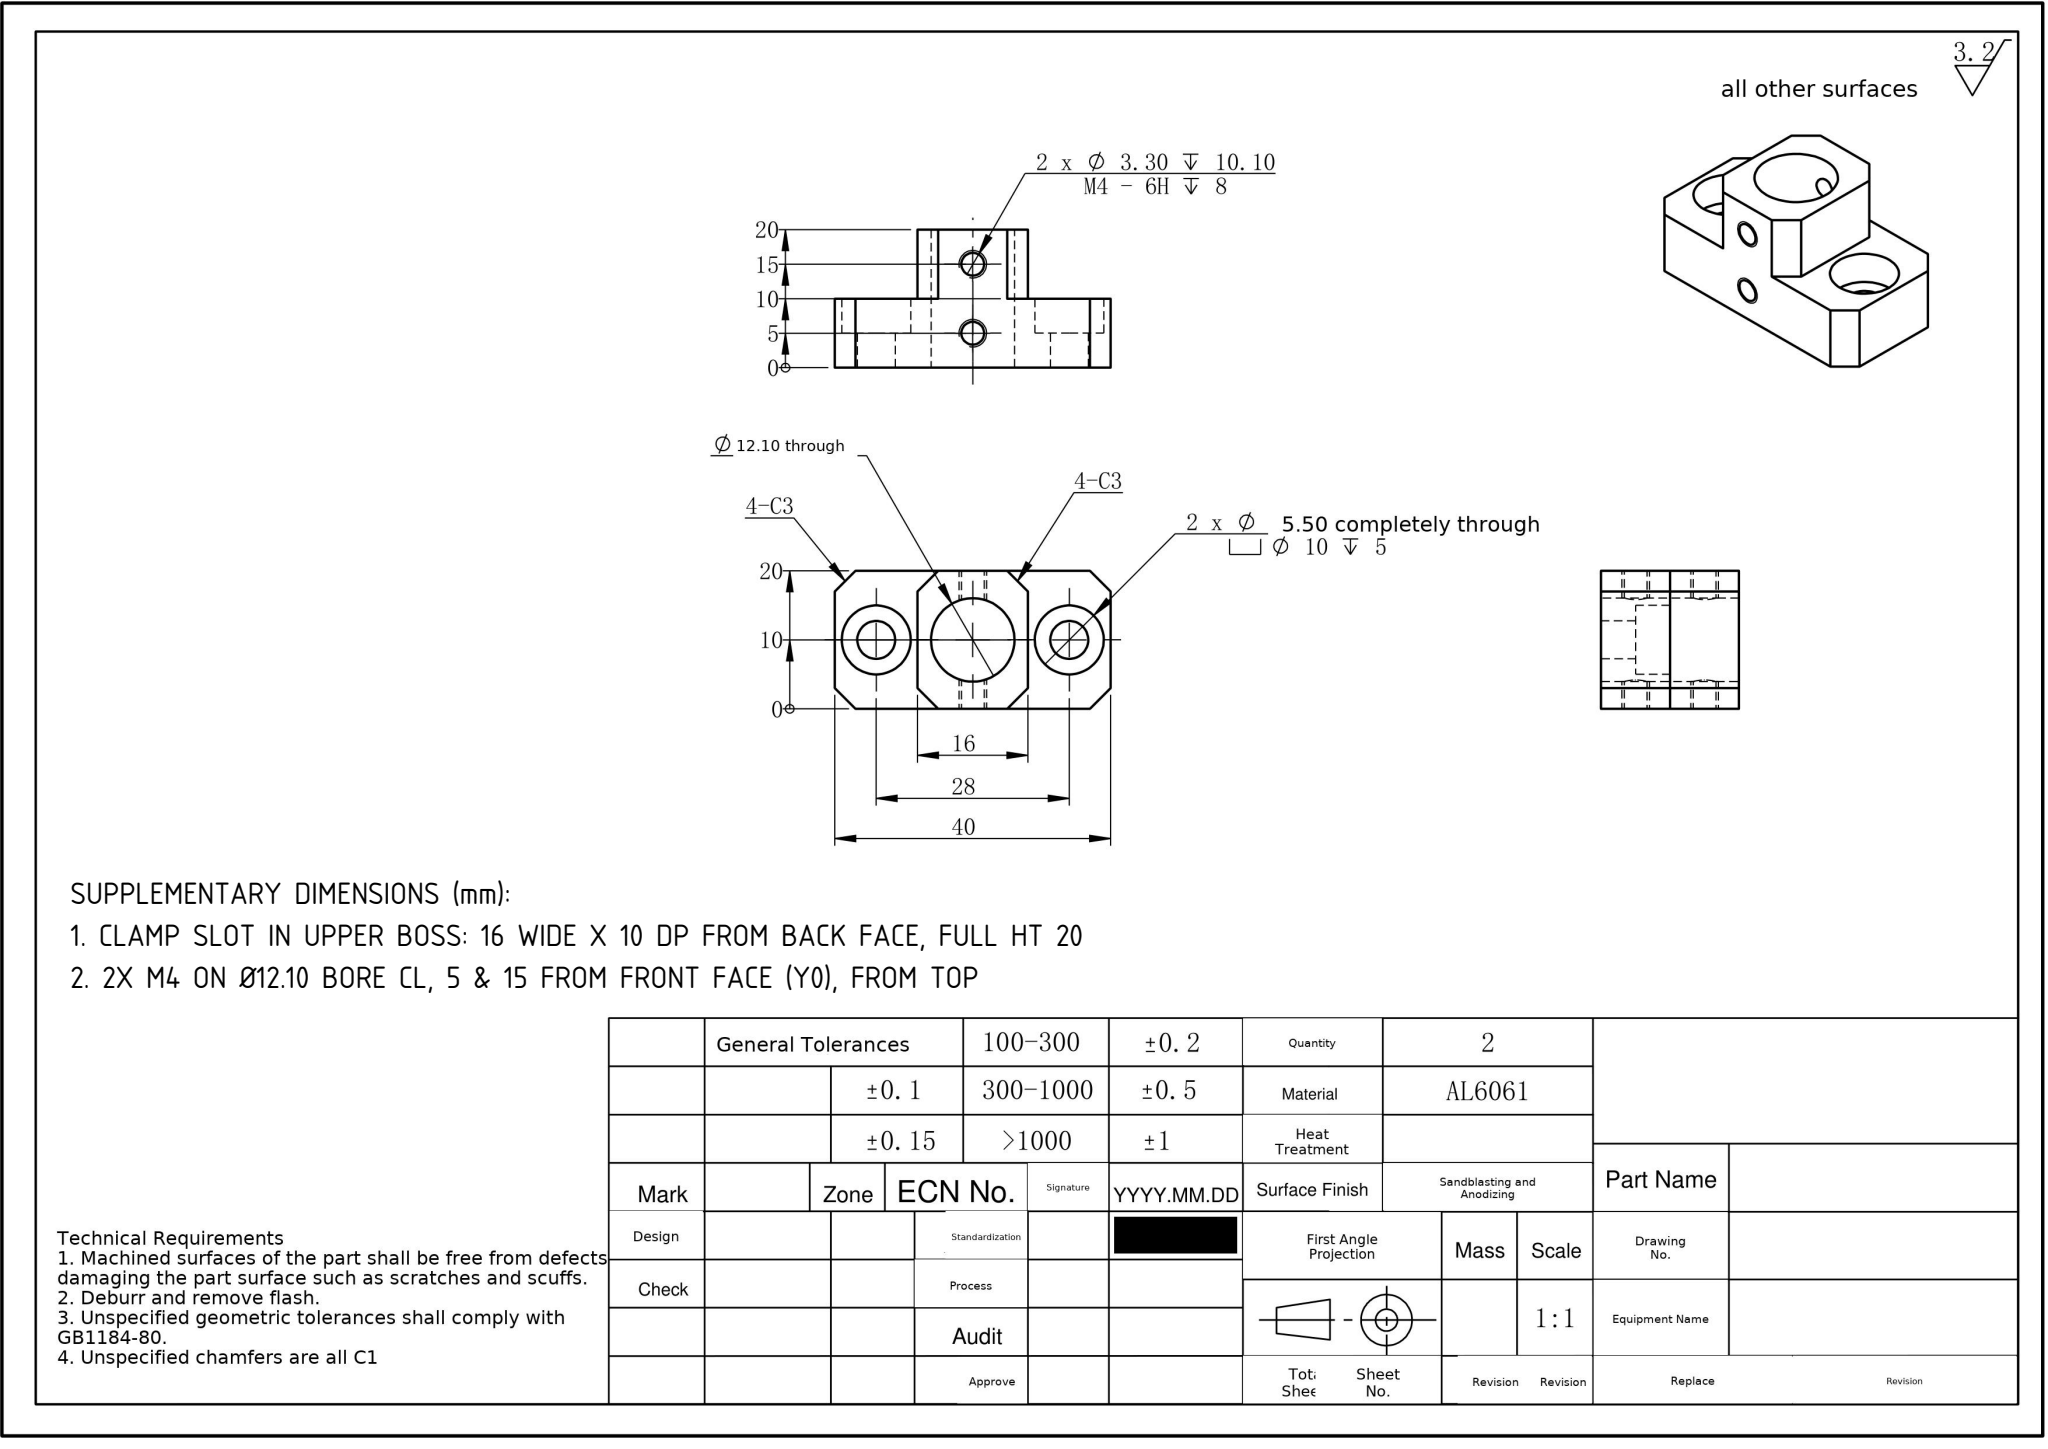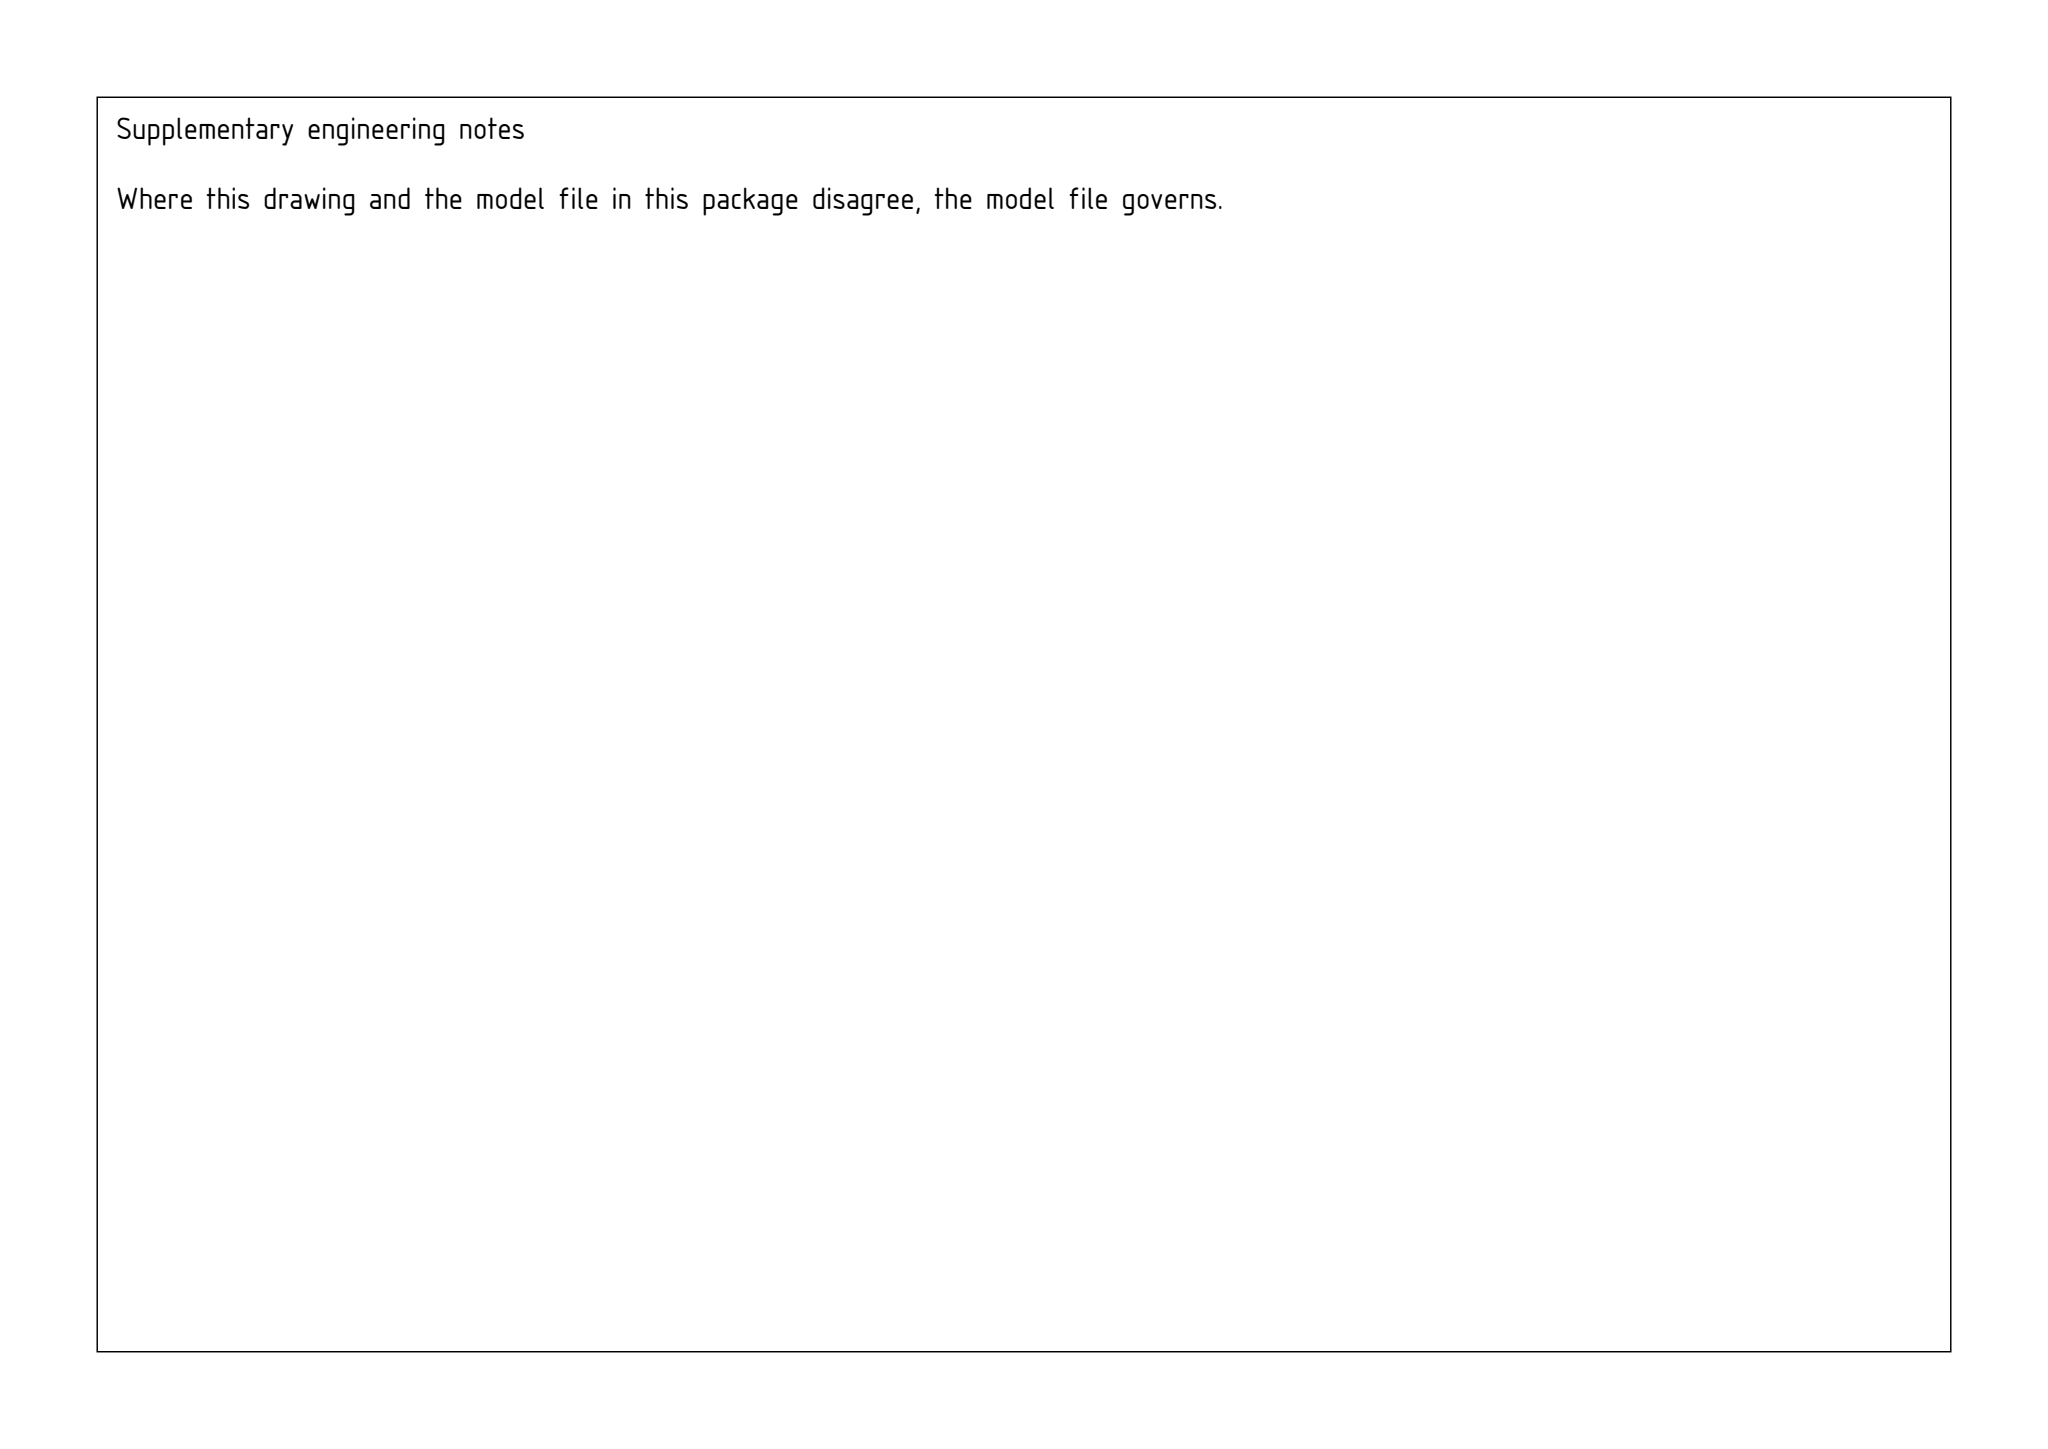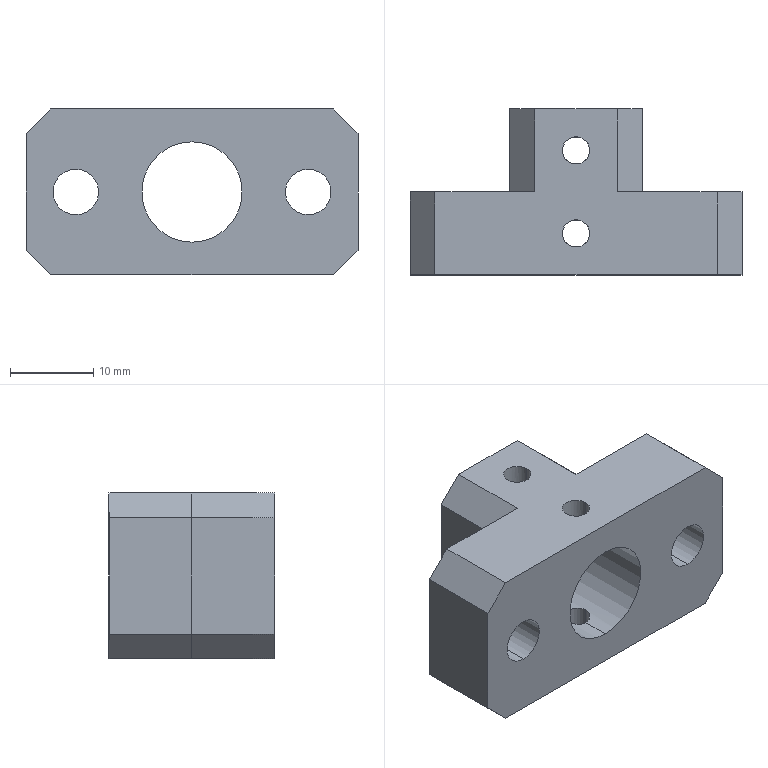Part | SolidWorks | mm | 1 solid | 38 faces | box 40 x 20 x 20 mm | volume 7380 mm3 | plane 20 | cylinder 18 | commonest cylinder face diameters 3.3 x8 10 x4 5.5 x4 12.1 x2
build123d program:
from build123d import *

# Parameters (mm, degrees)
SKETCH1_W                                       = 40
SKETCH1_H                                       = 20
SKETCH1_R                                       = 6.05
BOSS_EXTRUDE1_DEPTH                             = 20
SKETCH2_W                                       = 12
SKETCH2_H                                       = 10
CUT_EXTRUDE1_DEPTH                              = 20
CHAMFER1_SIZE                                   = 3
M4_TAPPED_HOLE1_AT_2_COUNT                      = 2
M4_TAPPED_HOLE1_AT_2_PITCH                      = 10
M5_HEX_SOCKET_HEAD_CAP_SCREW_CBORE1_D           = 5.5
M5_HEX_SOCKET_HEAD_CAP_SCREW_CBORE1_CBORE_D     = 10
M5_HEX_SOCKET_HEAD_CAP_SCREW_CBORE1_CBORE_DEPTH = 5


with BuildPart() as part:
    # Sketch1 → Boss-Extrude1 (new body)
    with BuildSketch(Plane(origin=(0, 0, 0), x_dir=(1, 0, 0), z_dir=(0, 1, 0))):
        Rectangle(SKETCH1_W, SKETCH1_H)
        with Locations(Location((0, 0, 0), (0, 0, 270))):
            Circle(SKETCH1_R, mode=Mode.SUBTRACT)
    extrude(amount=BOSS_EXTRUDE1_DEPTH)

    # Sketch2 → Cut-Extrude1 (cut)
    with BuildSketch(Plane.XY.offset(10)):
        with Locations((14, 15)):
            Rectangle(SKETCH2_W, SKETCH2_H)
        with Locations((-14, 15)):
            Rectangle(SKETCH2_W, SKETCH2_H)
    extrude(amount=-CUT_EXTRUDE1_DEPTH, mode=Mode.SUBTRACT)

    # Chamfer1
    chamfer1_edges = [part.edges().sort_by_distance(p)[0] for p in [
        (20, 5, 10),
        (20, 5, -10),
        (8, 15, 10),
        (8, 15, -10),
        (-20, 5, 10),
        (-20, 5, -10),
        (-8, 15, 10),
        (-8, 15, -10),
    ]]
    chamfer(chamfer1_edges, length=CHAMFER1_SIZE)

    # Sketch4 → M4 Tapped Hole1 (revolve, cut)
    with BuildSketch(Plane(origin=(0, 5, 10), x_dir=(0, -1, 0), z_dir=(1, 0, 0))):
        Polygon((0, 0), (0, 11.091), (1.65, 10.1), (1.65, 0), align=None)
    m4_tapped_hole1 = revolve(axis=Axis((0, 5, 16.35), (0, 0, -1)), mode=Mode.SUBTRACT)

    # M4 Tapped Hole1 at 2: M4 Tapped Hole1 ×2
    with Locations(*[(0, i * M4_TAPPED_HOLE1_AT_2_PITCH, 0) for i in range(1, M4_TAPPED_HOLE1_AT_2_COUNT)]):
        add(m4_tapped_hole1, mode=Mode.SUBTRACT)

    # M5 Hex Socket Head Cap Screw CBORE1 (through all)
    with Locations(Plane(origin=(0, 10, 0), x_dir=(1, 0, 0), z_dir=(0, 1, 0))):
        with Locations((14, 0), (-14, 0)):
            CounterBoreHole(M5_HEX_SOCKET_HEAD_CAP_SCREW_CBORE1_D / 2, M5_HEX_SOCKET_HEAD_CAP_SCREW_CBORE1_CBORE_D / 2, M5_HEX_SOCKET_HEAD_CAP_SCREW_CBORE1_CBORE_DEPTH)

    # Mirror1: M4 Tapped Hole1 across plane
    add(m4_tapped_hole1.mirror(Plane.XY), mode=Mode.SUBTRACT)

    # Mirror1 copy 1 sketch → Mirror1 copy 1 (revolve, cut)
    with BuildSketch(Plane(origin=(0, 15, -10), x_dir=(0, -1, 0), z_dir=(1, 0, 0))):
        Polygon((0, 0), (0, -11.091), (1.65, -10.1), (1.65, 0), align=None)
    revolve(axis=Axis((0, 15, -16.35), (0, 0, -1)), mode=Mode.SUBTRACT)


solid = part.part